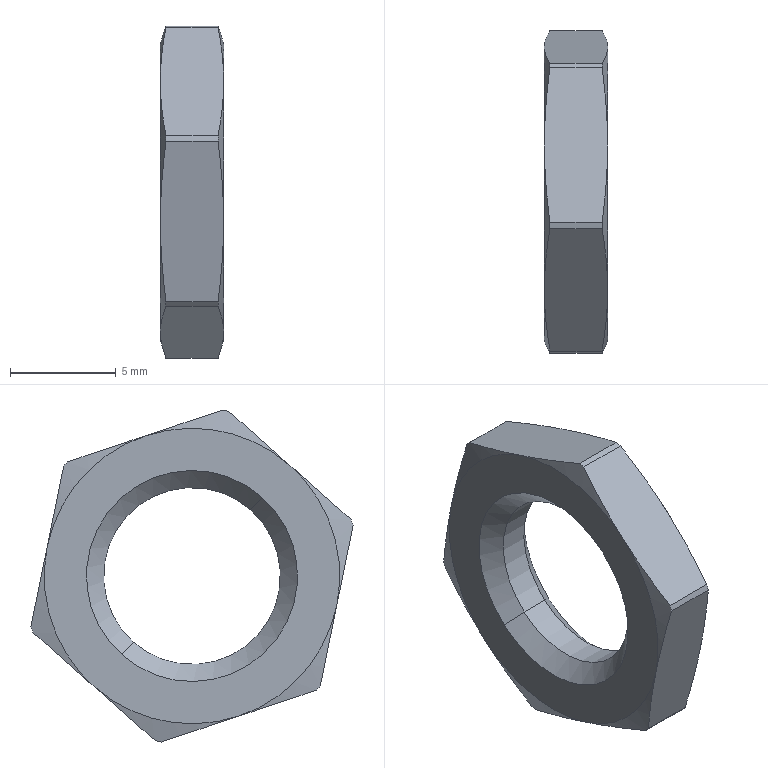Component | SolidWorks | SRK1010_nut_nut-1 | 1 solid | 32 faces | box 3 x 15.27 x 15.73 mm | volume 322 mm3 | cone 16 | cylinder 8 | plane 8 | commonest cylinder face diameters 16 x6 8.376 x2
STEP:
#1=COLOUR_RGB('',0.7922,0.8196,0.9333);
#2=FILL_AREA_STYLE_COLOUR('',#1);
#3=FILL_AREA_STYLE('',(#2));
#4=SURFACE_STYLE_FILL_AREA(#3);
#5=SURFACE_SIDE_STYLE('',(#4));
#6=SURFACE_STYLE_USAGE(.BOTH.,#5);
#7=PRESENTATION_STYLE_ASSIGNMENT((#6));
#8=CARTESIAN_POINT('',(-5.625,1.353,-4.032));
#9=VERTEX_POINT('',#8);
#10=CARTESIAN_POINT('',(-5.625,1.572,-4.278));
#11=VERTEX_POINT('',#10);
#12=CARTESIAN_POINT('',(-5.625,1.462,-4.155));
#13=DIRECTION('',(1.,-0.,-0.));
#14=DIRECTION('',(0.,0.6632,-0.7485));
#15=AXIS2_PLACEMENT_3D('',#12,#13,#14);
#16=CIRCLE('',#15,0.1649);
#17=EDGE_CURVE('',#9,#11,#16,.T.);
#18=ORIENTED_EDGE('',*,*,#17,.T.);
#19=CARTESIAN_POINT('',(-5.657,1.593,-4.302));
#20=VERTEX_POINT('',#19);
#21=CARTESIAN_POINT('',(-5.657,1.593,-4.302));
#22=DIRECTION('',(-0.7071,0.4689,-0.5292));
#23=VECTOR('',#22,39.37);
#24=LINE('',#21,#23);
#25=EDGE_CURVE('',#11,#20,#24,.T.);
#26=ORIENTED_EDGE('',*,*,#25,.T.);
#27=CARTESIAN_POINT('',(-5.657,1.332,-4.008));
#28=VERTEX_POINT('',#27);
#29=CARTESIAN_POINT('',(-5.657,1.462,-4.155));
#30=DIRECTION('',(1.,-0.,-0.));
#31=DIRECTION('',(0.,0.6632,-0.7485));
#32=AXIS2_PLACEMENT_3D('',#29,#30,#31);
#33=CIRCLE('',#32,0.1969);
#34=EDGE_CURVE('',#28,#20,#33,.T.);
#35=ORIENTED_EDGE('',*,*,#34,.F.);
#36=CARTESIAN_POINT('',(-5.657,1.332,-4.008));
#37=DIRECTION('',(-0.7071,-0.4689,0.5292));
#38=VECTOR('',#37,39.37);
#39=LINE('',#36,#38);
#40=EDGE_CURVE('',#9,#28,#39,.T.);
#41=ORIENTED_EDGE('',*,*,#40,.F.);
#42=EDGE_LOOP('',(#18,#26,#35,#41));
#43=FACE_OUTER_BOUND('',#42,.T.);
#44=CARTESIAN_POINT('',(-5.657,1.462,-4.155));
#45=DIRECTION('',(-1.,0.,0.));
#46=DIRECTION('',(0.,-0.6632,0.7485));
#47=AXIS2_PLACEMENT_3D('',#44,#45,#46);
#48=CONICAL_SURFACE('',#47,0.1969,0.7854);
#49=ADVANCED_FACE('',(#43),#48,.F.);
#50=ORIENTED_EDGE('',*,*,#17,.F.);
#51=CARTESIAN_POINT('',(-5.571,1.353,-4.032));
#52=VERTEX_POINT('',#51);
#53=CARTESIAN_POINT('',(-5.657,1.353,-4.032));
#54=DIRECTION('',(1.,-0.,-0.));
#55=VECTOR('',#54,39.37);
#56=LINE('',#53,#55);
#57=EDGE_CURVE('',#9,#52,#56,.T.);
#58=ORIENTED_EDGE('',*,*,#57,.T.);
#59=CARTESIAN_POINT('',(-5.571,1.572,-4.278));
#60=VERTEX_POINT('',#59);
#61=CARTESIAN_POINT('',(-5.571,1.462,-4.155));
#62=DIRECTION('',(1.,-0.,-0.));
#63=DIRECTION('',(0.,0.6632,-0.7485));
#64=AXIS2_PLACEMENT_3D('',#61,#62,#63);
#65=CIRCLE('',#64,0.1649);
#66=EDGE_CURVE('',#52,#60,#65,.T.);
#67=ORIENTED_EDGE('',*,*,#66,.T.);
#68=CARTESIAN_POINT('',(-5.657,1.572,-4.278));
#69=DIRECTION('',(1.,-0.,-0.));
#70=VECTOR('',#69,39.37);
#71=LINE('',#68,#70);
#72=EDGE_CURVE('',#11,#60,#71,.T.);
#73=ORIENTED_EDGE('',*,*,#72,.F.);
#74=EDGE_LOOP('',(#50,#58,#67,#73));
#75=FACE_OUTER_BOUND('',#74,.T.);
#76=CARTESIAN_POINT('',(-5.657,1.462,-4.155));
#77=DIRECTION('',(1.,-0.,-0.));
#78=DIRECTION('',(0.,0.6632,-0.7485));
#79=AXIS2_PLACEMENT_3D('',#76,#77,#78);
#80=CYLINDRICAL_SURFACE('',#79,0.1649);
#81=ADVANCED_FACE('',(#75),#80,.F.);
#82=ORIENTED_EDGE('',*,*,#66,.F.);
#83=CARTESIAN_POINT('',(-5.539,1.332,-4.008));
#84=VERTEX_POINT('',#83);
#85=CARTESIAN_POINT('',(-5.571,1.353,-4.032));
#86=DIRECTION('',(0.7071,-0.4689,0.5292));
#87=VECTOR('',#86,39.37);
#88=LINE('',#85,#87);
#89=EDGE_CURVE('',#52,#84,#88,.T.);
#90=ORIENTED_EDGE('',*,*,#89,.T.);
#91=CARTESIAN_POINT('',(-5.539,1.593,-4.302));
#92=VERTEX_POINT('',#91);
#93=CARTESIAN_POINT('',(-5.539,1.462,-4.155));
#94=DIRECTION('',(1.,-0.,-0.));
#95=DIRECTION('',(0.,0.6632,-0.7485));
#96=AXIS2_PLACEMENT_3D('',#93,#94,#95);
#97=CIRCLE('',#96,0.1969);
#98=EDGE_CURVE('',#84,#92,#97,.T.);
#99=ORIENTED_EDGE('',*,*,#98,.T.);
#100=CARTESIAN_POINT('',(-5.571,1.572,-4.278));
#101=DIRECTION('',(0.7071,0.4689,-0.5292));
#102=VECTOR('',#101,39.37);
#103=LINE('',#100,#102);
#104=EDGE_CURVE('',#60,#92,#103,.T.);
#105=ORIENTED_EDGE('',*,*,#104,.F.);
#106=EDGE_LOOP('',(#82,#90,#99,#105));
#107=FACE_OUTER_BOUND('',#106,.T.);
#108=CARTESIAN_POINT('',(-5.571,1.462,-4.155));
#109=DIRECTION('',(1.,-0.,-0.));
#110=DIRECTION('',(0.,0.6632,-0.7485));
#111=AXIS2_PLACEMENT_3D('',#108,#109,#110);
#112=CONICAL_SURFACE('',#111,0.1649,0.7854);
#113=ADVANCED_FACE('',(#107),#112,.F.);
#114=CARTESIAN_POINT('',(-5.539,1.645,-4.361));
#115=VERTEX_POINT('',#114);
#116=CARTESIAN_POINT('',(-5.539,1.732,-4.1));
#117=VERTEX_POINT('',#116);
#118=CARTESIAN_POINT('',(-5.539,1.462,-4.155));
#119=DIRECTION('',(1.,-0.,-0.));
#120=DIRECTION('',(0.,0.6632,-0.7485));
#121=AXIS2_PLACEMENT_3D('',#118,#119,#120);
#122=CIRCLE('',#121,0.2756);
#123=EDGE_CURVE('',#115,#117,#122,.T.);
#124=ORIENTED_EDGE('',*,*,#123,.T.);
#125=CARTESIAN_POINT('',(-5.539,1.549,-3.894));
#126=VERTEX_POINT('',#125);
#127=CARTESIAN_POINT('',(-5.539,1.462,-4.155));
#128=DIRECTION('',(1.,-0.,-0.));
#129=DIRECTION('',(0.,0.6632,-0.7485));
#130=AXIS2_PLACEMENT_3D('',#127,#128,#129);
#131=CIRCLE('',#130,0.2756);
#132=EDGE_CURVE('',#117,#126,#131,.T.);
#133=ORIENTED_EDGE('',*,*,#132,.T.);
#134=CARTESIAN_POINT('',(-5.539,1.279,-3.949));
#135=VERTEX_POINT('',#134);
#136=CARTESIAN_POINT('',(-5.539,1.462,-4.155));
#137=DIRECTION('',(1.,-0.,-0.));
#138=DIRECTION('',(0.,0.6632,-0.7485));
#139=AXIS2_PLACEMENT_3D('',#136,#137,#138);
#140=CIRCLE('',#139,0.2756);
#141=EDGE_CURVE('',#126,#135,#140,.T.);
#142=ORIENTED_EDGE('',*,*,#141,.T.);
#143=CARTESIAN_POINT('',(-5.539,1.192,-4.21));
#144=VERTEX_POINT('',#143);
#145=CARTESIAN_POINT('',(-5.539,1.462,-4.155));
#146=DIRECTION('',(1.,-0.,-0.));
#147=DIRECTION('',(0.,0.6632,-0.7485));
#148=AXIS2_PLACEMENT_3D('',#145,#146,#147);
#149=CIRCLE('',#148,0.2756);
#150=EDGE_CURVE('',#135,#144,#149,.T.);
#151=ORIENTED_EDGE('',*,*,#150,.T.);
#152=CARTESIAN_POINT('',(-5.539,1.375,-4.416));
#153=VERTEX_POINT('',#152);
#154=CARTESIAN_POINT('',(-5.539,1.462,-4.155));
#155=DIRECTION('',(1.,-0.,-0.));
#156=DIRECTION('',(0.,0.6632,-0.7485));
#157=AXIS2_PLACEMENT_3D('',#154,#155,#156);
#158=CIRCLE('',#157,0.2756);
#159=EDGE_CURVE('',#144,#153,#158,.T.);
#160=ORIENTED_EDGE('',*,*,#159,.T.);
#161=CARTESIAN_POINT('',(-5.539,1.462,-4.155));
#162=DIRECTION('',(1.,-0.,-0.));
#163=DIRECTION('',(0.,0.6632,-0.7485));
#164=AXIS2_PLACEMENT_3D('',#161,#162,#163);
#165=CIRCLE('',#164,0.2756);
#166=EDGE_CURVE('',#153,#115,#165,.T.);
#167=ORIENTED_EDGE('',*,*,#166,.T.);
#168=EDGE_LOOP('',(#124,#133,#142,#151,#160,#167));
#169=FACE_OUTER_BOUND('',#168,.T.);
#170=CARTESIAN_POINT('',(-5.539,1.462,-4.155));
#171=DIRECTION('',(1.,-0.,-0.));
#172=DIRECTION('',(0.,0.6632,-0.7485));
#173=AXIS2_PLACEMENT_3D('',#170,#171,#172);
#174=CIRCLE('',#173,0.1969);
#175=EDGE_CURVE('',#92,#84,#174,.T.);
#176=ORIENTED_EDGE('',*,*,#175,.F.);
#177=ORIENTED_EDGE('',*,*,#98,.F.);
#178=EDGE_LOOP('',(#176,#177));
#179=FACE_BOUND('',#178,.T.);
#180=CARTESIAN_POINT('',(-5.539,1.462,-4.155));
#181=DIRECTION('',(-1.,0.,0.));
#182=DIRECTION('',(-0.,-0.6632,0.7485));
#183=AXIS2_PLACEMENT_3D('',#180,#181,#182);
#184=PLANE('',#183);
#185=ADVANCED_FACE('',(#169,#179),#184,.F.);
#186=CARTESIAN_POINT('',(-5.657,1.645,-4.361));
#187=VERTEX_POINT('',#186);
#188=CARTESIAN_POINT('',(-5.657,1.732,-4.1));
#189=VERTEX_POINT('',#188);
#190=CARTESIAN_POINT('',(-5.657,1.462,-4.155));
#191=DIRECTION('',(1.,-0.,-0.));
#192=DIRECTION('',(0.,0.6632,-0.7485));
#193=AXIS2_PLACEMENT_3D('',#190,#191,#192);
#194=CIRCLE('',#193,0.2756);
#195=EDGE_CURVE('',#187,#189,#194,.T.);
#196=ORIENTED_EDGE('',*,*,#195,.F.);
#197=CARTESIAN_POINT('',(-5.657,1.375,-4.416));
#198=VERTEX_POINT('',#197);
#199=CARTESIAN_POINT('',(-5.657,1.462,-4.155));
#200=DIRECTION('',(1.,-0.,-0.));
#201=DIRECTION('',(0.,0.6632,-0.7485));
#202=AXIS2_PLACEMENT_3D('',#199,#200,#201);
#203=CIRCLE('',#202,0.2756);
#204=EDGE_CURVE('',#198,#187,#203,.T.);
#205=ORIENTED_EDGE('',*,*,#204,.F.);
#206=CARTESIAN_POINT('',(-5.657,1.192,-4.21));
#207=VERTEX_POINT('',#206);
#208=CARTESIAN_POINT('',(-5.657,1.462,-4.155));
#209=DIRECTION('',(1.,-0.,-0.));
#210=DIRECTION('',(0.,0.6632,-0.7485));
#211=AXIS2_PLACEMENT_3D('',#208,#209,#210);
#212=CIRCLE('',#211,0.2756);
#213=EDGE_CURVE('',#207,#198,#212,.T.);
#214=ORIENTED_EDGE('',*,*,#213,.F.);
#215=CARTESIAN_POINT('',(-5.657,1.279,-3.949));
#216=VERTEX_POINT('',#215);
#217=CARTESIAN_POINT('',(-5.657,1.462,-4.155));
#218=DIRECTION('',(1.,-0.,-0.));
#219=DIRECTION('',(0.,0.6632,-0.7485));
#220=AXIS2_PLACEMENT_3D('',#217,#218,#219);
#221=CIRCLE('',#220,0.2756);
#222=EDGE_CURVE('',#216,#207,#221,.T.);
#223=ORIENTED_EDGE('',*,*,#222,.F.);
#224=CARTESIAN_POINT('',(-5.657,1.549,-3.894));
#225=VERTEX_POINT('',#224);
#226=CARTESIAN_POINT('',(-5.657,1.462,-4.155));
#227=DIRECTION('',(1.,-0.,-0.));
#228=DIRECTION('',(0.,0.6632,-0.7485));
#229=AXIS2_PLACEMENT_3D('',#226,#227,#228);
#230=CIRCLE('',#229,0.2756);
#231=EDGE_CURVE('',#225,#216,#230,.T.);
#232=ORIENTED_EDGE('',*,*,#231,.F.);
#233=CARTESIAN_POINT('',(-5.657,1.462,-4.155));
#234=DIRECTION('',(1.,-0.,-0.));
#235=DIRECTION('',(0.,0.6632,-0.7485));
#236=AXIS2_PLACEMENT_3D('',#233,#234,#235);
#237=CIRCLE('',#236,0.2756);
#238=EDGE_CURVE('',#189,#225,#237,.T.);
#239=ORIENTED_EDGE('',*,*,#238,.F.);
#240=EDGE_LOOP('',(#196,#205,#214,#223,#232,#239));
#241=FACE_OUTER_BOUND('',#240,.T.);
#242=ORIENTED_EDGE('',*,*,#34,.T.);
#243=CARTESIAN_POINT('',(-5.657,1.462,-4.155));
#244=DIRECTION('',(1.,-0.,-0.));
#245=DIRECTION('',(0.,0.6632,-0.7485));
#246=AXIS2_PLACEMENT_3D('',#243,#244,#245);
#247=CIRCLE('',#246,0.1969);
#248=EDGE_CURVE('',#20,#28,#247,.T.);
#249=ORIENTED_EDGE('',*,*,#248,.T.);
#250=EDGE_LOOP('',(#242,#249));
#251=FACE_BOUND('',#250,.T.);
#252=CARTESIAN_POINT('',(-5.657,1.669,-3.972));
#253=DIRECTION('',(1.,-0.,-0.));
#254=DIRECTION('',(0.,0.6632,-0.7485));
#255=AXIS2_PLACEMENT_3D('',#252,#253,#254);
#256=PLANE('',#255);
#257=ADVANCED_FACE('',(#241,#251),#256,.F.);
#258=CARTESIAN_POINT('',(-5.55,1.223,-4.36));
#259=VERTEX_POINT('',#258);
#260=CARTESIAN_POINT('',(-5.55,1.223,-4.36));
#261=CARTESIAN_POINT('',(-5.543,1.213,-4.31));
#262=CARTESIAN_POINT('',(-5.539,1.202,-4.26));
#263=CARTESIAN_POINT('',(-5.539,1.192,-4.21));
#264=B_SPLINE_CURVE_WITH_KNOTS('',3,(#260,#261,#262,#263),.UNSPECIFIED.,.F.,.F.,(4,4),(0.00000154,0.003875),.UNSPECIFIED.);
#265=EDGE_CURVE('',#259,#144,#264,.T.);
#266=ORIENTED_EDGE('',*,*,#265,.F.);
#267=CARTESIAN_POINT('',(-5.55,1.23,-4.368));
#268=VERTEX_POINT('',#267);
#269=CARTESIAN_POINT('',(-5.55,1.462,-4.155));
#270=DIRECTION('',(1.,-0.,-0.));
#271=DIRECTION('',(0.,0.6632,-0.7485));
#272=AXIS2_PLACEMENT_3D('',#269,#270,#271);
#273=CIRCLE('',#272,0.315);
#274=EDGE_CURVE('',#259,#268,#273,.T.);
#275=ORIENTED_EDGE('',*,*,#274,.T.);
#276=CARTESIAN_POINT('',(-5.539,1.375,-4.416));
#277=CARTESIAN_POINT('',(-5.539,1.327,-4.4));
#278=CARTESIAN_POINT('',(-5.543,1.279,-4.384));
#279=CARTESIAN_POINT('',(-5.55,1.23,-4.368));
#280=B_SPLINE_CURVE_WITH_KNOTS('',3,(#276,#277,#278,#279),.UNSPECIFIED.,.F.,.F.,(4,4),(0.003875,0.007748),.UNSPECIFIED.);
#281=EDGE_CURVE('',#153,#268,#280,.T.);
#282=ORIENTED_EDGE('',*,*,#281,.F.);
#283=ORIENTED_EDGE('',*,*,#159,.F.);
#284=EDGE_LOOP('',(#266,#275,#282,#283));
#285=FACE_OUTER_BOUND('',#284,.T.);
#286=CARTESIAN_POINT('',(-5.55,1.462,-4.155));
#287=DIRECTION('',(-1.,0.,0.));
#288=DIRECTION('',(0.,-0.6632,0.7485));
#289=AXIS2_PLACEMENT_3D('',#286,#287,#288);
#290=CONICAL_SURFACE('',#289,0.315,1.309);
#291=ADVANCED_FACE('',(#285),#290,.T.);
#292=CARTESIAN_POINT('',(-5.55,1.162,-4.061));
#293=VERTEX_POINT('',#292);
#294=CARTESIAN_POINT('',(-5.539,1.192,-4.21));
#295=CARTESIAN_POINT('',(-5.539,1.182,-4.16));
#296=CARTESIAN_POINT('',(-5.543,1.172,-4.111));
#297=CARTESIAN_POINT('',(-5.55,1.162,-4.061));
#298=B_SPLINE_CURVE_WITH_KNOTS('',3,(#294,#295,#296,#297),.UNSPECIFIED.,.F.,.F.,(4,4),(0.003875,0.007748),.UNSPECIFIED.);
#299=EDGE_CURVE('',#144,#293,#298,.T.);
#300=ORIENTED_EDGE('',*,*,#299,.F.);
#301=ORIENTED_EDGE('',*,*,#150,.F.);
#302=CARTESIAN_POINT('',(-5.55,1.165,-4.05));
#303=VERTEX_POINT('',#302);
#304=CARTESIAN_POINT('',(-5.55,1.165,-4.05));
#305=CARTESIAN_POINT('',(-5.546,1.184,-4.033));
#306=CARTESIAN_POINT('',(-5.544,1.203,-4.016));
#307=CARTESIAN_POINT('',(-5.54,1.241,-3.982));
#308=CARTESIAN_POINT('',(-5.539,1.26,-3.966));
#309=CARTESIAN_POINT('',(-5.539,1.279,-3.949));
#310=B_SPLINE_CURVE_WITH_KNOTS('',3,(#304,#305,#306,#307,#308,#309),.UNSPECIFIED.,.F.,.F.,(4,2,4),(0.006929,0.008875,0.01082),.UNSPECIFIED.);
#311=EDGE_CURVE('',#303,#135,#310,.T.);
#312=ORIENTED_EDGE('',*,*,#311,.F.);
#313=CARTESIAN_POINT('',(-5.55,1.462,-4.155));
#314=DIRECTION('',(1.,-0.,-0.));
#315=DIRECTION('',(0.,0.6632,-0.7485));
#316=AXIS2_PLACEMENT_3D('',#313,#314,#315);
#317=CIRCLE('',#316,0.315);
#318=EDGE_CURVE('',#303,#293,#317,.T.);
#319=ORIENTED_EDGE('',*,*,#318,.T.);
#320=EDGE_LOOP('',(#300,#301,#312,#319));
#321=FACE_OUTER_BOUND('',#320,.T.);
#322=CARTESIAN_POINT('',(-5.55,1.462,-4.155));
#323=DIRECTION('',(-1.,0.,0.));
#324=DIRECTION('',(0.,-0.6632,0.7485));
#325=AXIS2_PLACEMENT_3D('',#322,#323,#324);
#326=CONICAL_SURFACE('',#325,0.315,1.309);
#327=ADVANCED_FACE('',(#321),#326,.T.);
#328=CARTESIAN_POINT('',(-5.55,1.394,-3.848));
#329=VERTEX_POINT('',#328);
#330=CARTESIAN_POINT('',(-5.539,1.279,-3.949));
#331=CARTESIAN_POINT('',(-5.539,1.318,-3.915));
#332=CARTESIAN_POINT('',(-5.543,1.356,-3.881));
#333=CARTESIAN_POINT('',(-5.55,1.394,-3.848));
#334=B_SPLINE_CURVE_WITH_KNOTS('',3,(#330,#331,#332,#333),.UNSPECIFIED.,.F.,.F.,(4,4),(0.01082,0.01473),.UNSPECIFIED.);
#335=EDGE_CURVE('',#135,#329,#334,.T.);
#336=ORIENTED_EDGE('',*,*,#335,.F.);
#337=ORIENTED_EDGE('',*,*,#141,.F.);
#338=CARTESIAN_POINT('',(-5.55,1.405,-3.845));
#339=VERTEX_POINT('',#338);
#340=CARTESIAN_POINT('',(-5.55,1.405,-3.845));
#341=CARTESIAN_POINT('',(-5.543,1.453,-3.861));
#342=CARTESIAN_POINT('',(-5.539,1.501,-3.877));
#343=CARTESIAN_POINT('',(-5.539,1.549,-3.894));
#344=B_SPLINE_CURVE_WITH_KNOTS('',3,(#340,#341,#342,#343),.UNSPECIFIED.,.F.,.F.,(4,4),(0.00000154,0.003875),.UNSPECIFIED.);
#345=EDGE_CURVE('',#339,#126,#344,.T.);
#346=ORIENTED_EDGE('',*,*,#345,.F.);
#347=CARTESIAN_POINT('',(-5.55,1.462,-4.155));
#348=DIRECTION('',(1.,-0.,-0.));
#349=DIRECTION('',(0.,0.6632,-0.7485));
#350=AXIS2_PLACEMENT_3D('',#347,#348,#349);
#351=CIRCLE('',#350,0.315);
#352=EDGE_CURVE('',#339,#329,#351,.T.);
#353=ORIENTED_EDGE('',*,*,#352,.T.);
#354=EDGE_LOOP('',(#336,#337,#346,#353));
#355=FACE_OUTER_BOUND('',#354,.T.);
#356=CARTESIAN_POINT('',(-5.55,1.462,-4.155));
#357=DIRECTION('',(-1.,0.,0.));
#358=DIRECTION('',(0.,-0.6632,0.7485));
#359=AXIS2_PLACEMENT_3D('',#356,#357,#358);
#360=CONICAL_SURFACE('',#359,0.315,1.309);
#361=ADVANCED_FACE('',(#355),#360,.T.);
#362=CARTESIAN_POINT('',(-5.55,1.694,-3.942));
#363=VERTEX_POINT('',#362);
#364=CARTESIAN_POINT('',(-5.539,1.549,-3.894));
#365=CARTESIAN_POINT('',(-5.539,1.598,-3.91));
#366=CARTESIAN_POINT('',(-5.543,1.646,-3.926));
#367=CARTESIAN_POINT('',(-5.55,1.694,-3.942));
#368=B_SPLINE_CURVE_WITH_KNOTS('',3,(#364,#365,#366,#367),.UNSPECIFIED.,.F.,.F.,(4,4),(0.003875,0.007748),.UNSPECIFIED.);
#369=EDGE_CURVE('',#126,#363,#368,.T.);
#370=ORIENTED_EDGE('',*,*,#369,.F.);
#371=ORIENTED_EDGE('',*,*,#132,.F.);
#372=CARTESIAN_POINT('',(-5.55,1.702,-3.95));
#373=VERTEX_POINT('',#372);
#374=CARTESIAN_POINT('',(-5.55,1.702,-3.95));
#375=CARTESIAN_POINT('',(-5.543,1.712,-4.));
#376=CARTESIAN_POINT('',(-5.539,1.722,-4.05));
#377=CARTESIAN_POINT('',(-5.539,1.732,-4.1));
#378=B_SPLINE_CURVE_WITH_KNOTS('',3,(#374,#375,#376,#377),.UNSPECIFIED.,.F.,.F.,(4,4),(0.00000154,0.003875),.UNSPECIFIED.);
#379=EDGE_CURVE('',#373,#117,#378,.T.);
#380=ORIENTED_EDGE('',*,*,#379,.F.);
#381=CARTESIAN_POINT('',(-5.55,1.462,-4.155));
#382=DIRECTION('',(1.,-0.,-0.));
#383=DIRECTION('',(0.,0.6632,-0.7485));
#384=AXIS2_PLACEMENT_3D('',#381,#382,#383);
#385=CIRCLE('',#384,0.315);
#386=EDGE_CURVE('',#373,#363,#385,.T.);
#387=ORIENTED_EDGE('',*,*,#386,.T.);
#388=EDGE_LOOP('',(#370,#371,#380,#387));
#389=FACE_OUTER_BOUND('',#388,.T.);
#390=CARTESIAN_POINT('',(-5.55,1.462,-4.155));
#391=DIRECTION('',(-1.,0.,0.));
#392=DIRECTION('',(0.,-0.6632,0.7485));
#393=AXIS2_PLACEMENT_3D('',#390,#391,#392);
#394=CONICAL_SURFACE('',#393,0.315,1.309);
#395=ADVANCED_FACE('',(#389),#394,.T.);
#396=CARTESIAN_POINT('',(-5.55,1.763,-4.249));
#397=VERTEX_POINT('',#396);
#398=CARTESIAN_POINT('',(-5.539,1.732,-4.1));
#399=CARTESIAN_POINT('',(-5.539,1.742,-4.15));
#400=CARTESIAN_POINT('',(-5.543,1.753,-4.199));
#401=CARTESIAN_POINT('',(-5.55,1.763,-4.249));
#402=B_SPLINE_CURVE_WITH_KNOTS('',3,(#398,#399,#400,#401),.UNSPECIFIED.,.F.,.F.,(4,4),(0.003875,0.007748),.UNSPECIFIED.);
#403=EDGE_CURVE('',#117,#397,#402,.T.);
#404=ORIENTED_EDGE('',*,*,#403,.F.);
#405=ORIENTED_EDGE('',*,*,#123,.F.);
#406=CARTESIAN_POINT('',(-5.55,1.759,-4.26));
#407=VERTEX_POINT('',#406);
#408=CARTESIAN_POINT('',(-5.55,1.759,-4.26));
#409=CARTESIAN_POINT('',(-5.543,1.721,-4.294));
#410=CARTESIAN_POINT('',(-5.539,1.683,-4.327));
#411=CARTESIAN_POINT('',(-5.539,1.645,-4.361));
#412=B_SPLINE_CURVE_WITH_KNOTS('',3,(#408,#409,#410,#411),.UNSPECIFIED.,.F.,.F.,(4,4),(0.01554,0.01944),.UNSPECIFIED.);
#413=EDGE_CURVE('',#407,#115,#412,.T.);
#414=ORIENTED_EDGE('',*,*,#413,.F.);
#415=CARTESIAN_POINT('',(-5.55,1.462,-4.155));
#416=DIRECTION('',(1.,-0.,-0.));
#417=DIRECTION('',(0.,0.6632,-0.7485));
#418=AXIS2_PLACEMENT_3D('',#415,#416,#417);
#419=CIRCLE('',#418,0.315);
#420=EDGE_CURVE('',#407,#397,#419,.T.);
#421=ORIENTED_EDGE('',*,*,#420,.T.);
#422=EDGE_LOOP('',(#404,#405,#414,#421));
#423=FACE_OUTER_BOUND('',#422,.T.);
#424=CARTESIAN_POINT('',(-5.55,1.462,-4.155));
#425=DIRECTION('',(-1.,0.,0.));
#426=DIRECTION('',(0.,-0.6632,0.7485));
#427=AXIS2_PLACEMENT_3D('',#424,#425,#426);
#428=CONICAL_SURFACE('',#427,0.315,1.309);
#429=ADVANCED_FACE('',(#423),#428,.T.);
#430=CARTESIAN_POINT('',(-5.55,1.531,-4.462));
#431=VERTEX_POINT('',#430);
#432=CARTESIAN_POINT('',(-5.539,1.645,-4.361));
#433=CARTESIAN_POINT('',(-5.539,1.626,-4.378));
#434=CARTESIAN_POINT('',(-5.54,1.607,-4.395));
#435=CARTESIAN_POINT('',(-5.544,1.569,-4.429));
#436=CARTESIAN_POINT('',(-5.546,1.55,-4.446));
#437=CARTESIAN_POINT('',(-5.55,1.531,-4.462));
#438=B_SPLINE_CURVE_WITH_KNOTS('',3,(#432,#433,#434,#435,#436,#437),.UNSPECIFIED.,.F.,.F.,(4,2,4),(0.01944,0.02138,0.02332),.UNSPECIFIED.);
#439=EDGE_CURVE('',#115,#431,#438,.T.);
#440=ORIENTED_EDGE('',*,*,#439,.F.);
#441=ORIENTED_EDGE('',*,*,#166,.F.);
#442=CARTESIAN_POINT('',(-5.55,1.52,-4.465));
#443=VERTEX_POINT('',#442);
#444=CARTESIAN_POINT('',(-5.55,1.52,-4.465));
#445=CARTESIAN_POINT('',(-5.543,1.471,-4.449));
#446=CARTESIAN_POINT('',(-5.539,1.423,-4.432));
#447=CARTESIAN_POINT('',(-5.539,1.375,-4.416));
#448=B_SPLINE_CURVE_WITH_KNOTS('',3,(#444,#445,#446,#447),.UNSPECIFIED.,.F.,.F.,(4,4),(0.00000154,0.003875),.UNSPECIFIED.);
#449=EDGE_CURVE('',#443,#153,#448,.T.);
#450=ORIENTED_EDGE('',*,*,#449,.F.);
#451=CARTESIAN_POINT('',(-5.55,1.462,-4.155));
#452=DIRECTION('',(1.,-0.,-0.));
#453=DIRECTION('',(0.,0.6632,-0.7485));
#454=AXIS2_PLACEMENT_3D('',#451,#452,#453);
#455=CIRCLE('',#454,0.315);
#456=EDGE_CURVE('',#443,#431,#455,.T.);
#457=ORIENTED_EDGE('',*,*,#456,.T.);
#458=EDGE_LOOP('',(#440,#441,#450,#457));
#459=FACE_OUTER_BOUND('',#458,.T.);
#460=CARTESIAN_POINT('',(-5.55,1.462,-4.155));
#461=DIRECTION('',(-1.,0.,0.));
#462=DIRECTION('',(0.,-0.6632,0.7485));
#463=AXIS2_PLACEMENT_3D('',#460,#461,#462);
#464=CONICAL_SURFACE('',#463,0.315,1.309);
#465=ADVANCED_FACE('',(#459),#464,.T.);
#466=CARTESIAN_POINT('',(-5.647,1.223,-4.36));
#467=VERTEX_POINT('',#466);
#468=CARTESIAN_POINT('',(-5.657,1.223,-4.36));
#469=DIRECTION('',(1.,-0.,-0.));
#470=VECTOR('',#469,39.37);
#471=LINE('',#468,#470);
#472=EDGE_CURVE('',#467,#259,#471,.T.);
#473=ORIENTED_EDGE('',*,*,#472,.F.);
#474=CARTESIAN_POINT('',(-5.647,1.23,-4.368));
#475=VERTEX_POINT('',#474);
#476=CARTESIAN_POINT('',(-5.647,1.462,-4.155));
#477=DIRECTION('',(1.,-0.,-0.));
#478=DIRECTION('',(0.,0.6632,-0.7485));
#479=AXIS2_PLACEMENT_3D('',#476,#477,#478);
#480=CIRCLE('',#479,0.315);
#481=EDGE_CURVE('',#467,#475,#480,.T.);
#482=ORIENTED_EDGE('',*,*,#481,.T.);
#483=CARTESIAN_POINT('',(-5.657,1.23,-4.368));
#484=DIRECTION('',(-1.,0.,0.));
#485=VECTOR('',#484,39.37);
#486=LINE('',#483,#485);
#487=EDGE_CURVE('',#268,#475,#486,.T.);
#488=ORIENTED_EDGE('',*,*,#487,.F.);
#489=ORIENTED_EDGE('',*,*,#274,.F.);
#490=EDGE_LOOP('',(#473,#482,#488,#489));
#491=FACE_OUTER_BOUND('',#490,.T.);
#492=CARTESIAN_POINT('',(-5.657,1.462,-4.155));
#493=DIRECTION('',(1.,-0.,-0.));
#494=DIRECTION('',(0.,0.6632,-0.7485));
#495=AXIS2_PLACEMENT_3D('',#492,#493,#494);
#496=CYLINDRICAL_SURFACE('',#495,0.315);
#497=ADVANCED_FACE('',(#491),#496,.T.);
#498=CARTESIAN_POINT('',(-5.647,1.162,-4.061));
#499=VERTEX_POINT('',#498);
#500=CARTESIAN_POINT('',(-5.657,1.162,-4.061));
#501=DIRECTION('',(-1.,0.,0.));
#502=VECTOR('',#501,39.37);
#503=LINE('',#500,#502);
#504=EDGE_CURVE('',#293,#499,#503,.T.);
#505=ORIENTED_EDGE('',*,*,#504,.F.);
#506=ORIENTED_EDGE('',*,*,#318,.F.);
#507=CARTESIAN_POINT('',(-5.647,1.165,-4.05));
#508=VERTEX_POINT('',#507);
#509=CARTESIAN_POINT('',(-5.657,1.165,-4.05));
#510=DIRECTION('',(1.,-0.,-0.));
#511=VECTOR('',#510,39.37);
#512=LINE('',#509,#511);
#513=EDGE_CURVE('',#508,#303,#512,.T.);
#514=ORIENTED_EDGE('',*,*,#513,.F.);
#515=CARTESIAN_POINT('',(-5.647,1.462,-4.155));
#516=DIRECTION('',(1.,-0.,-0.));
#517=DIRECTION('',(0.,0.6632,-0.7485));
#518=AXIS2_PLACEMENT_3D('',#515,#516,#517);
#519=CIRCLE('',#518,0.315);
#520=EDGE_CURVE('',#508,#499,#519,.T.);
#521=ORIENTED_EDGE('',*,*,#520,.T.);
#522=EDGE_LOOP('',(#505,#506,#514,#521));
#523=FACE_OUTER_BOUND('',#522,.T.);
#524=CARTESIAN_POINT('',(-5.657,1.462,-4.155));
#525=DIRECTION('',(1.,-0.,-0.));
#526=DIRECTION('',(0.,0.6632,-0.7485));
#527=AXIS2_PLACEMENT_3D('',#524,#525,#526);
#528=CYLINDRICAL_SURFACE('',#527,0.315);
#529=ADVANCED_FACE('',(#523),#528,.T.);
#530=CARTESIAN_POINT('',(-5.647,1.394,-3.848));
#531=VERTEX_POINT('',#530);
#532=CARTESIAN_POINT('',(-5.657,1.394,-3.848));
#533=DIRECTION('',(-1.,0.,0.));
#534=VECTOR('',#533,39.37);
#535=LINE('',#532,#534);
#536=EDGE_CURVE('',#329,#531,#535,.T.);
#537=ORIENTED_EDGE('',*,*,#536,.F.);
#538=ORIENTED_EDGE('',*,*,#352,.F.);
#539=CARTESIAN_POINT('',(-5.647,1.405,-3.845));
#540=VERTEX_POINT('',#539);
#541=CARTESIAN_POINT('',(-5.657,1.405,-3.845));
#542=DIRECTION('',(1.,-0.,-0.));
#543=VECTOR('',#542,39.37);
#544=LINE('',#541,#543);
#545=EDGE_CURVE('',#540,#339,#544,.T.);
#546=ORIENTED_EDGE('',*,*,#545,.F.);
#547=CARTESIAN_POINT('',(-5.647,1.462,-4.155));
#548=DIRECTION('',(1.,-0.,-0.));
#549=DIRECTION('',(0.,0.6632,-0.7485));
#550=AXIS2_PLACEMENT_3D('',#547,#548,#549);
#551=CIRCLE('',#550,0.315);
#552=EDGE_CURVE('',#540,#531,#551,.T.);
#553=ORIENTED_EDGE('',*,*,#552,.T.);
#554=EDGE_LOOP('',(#537,#538,#546,#553));
#555=FACE_OUTER_BOUND('',#554,.T.);
#556=CARTESIAN_POINT('',(-5.657,1.462,-4.155));
#557=DIRECTION('',(1.,-0.,-0.));
#558=DIRECTION('',(0.,0.6632,-0.7485));
#559=AXIS2_PLACEMENT_3D('',#556,#557,#558);
#560=CYLINDRICAL_SURFACE('',#559,0.315);
#561=ADVANCED_FACE('',(#555),#560,.T.);
#562=CARTESIAN_POINT('',(-5.647,1.694,-3.942));
#563=VERTEX_POINT('',#562);
#564=CARTESIAN_POINT('',(-5.657,1.694,-3.942));
#565=DIRECTION('',(-1.,0.,0.));
#566=VECTOR('',#565,39.37);
#567=LINE('',#564,#566);
#568=EDGE_CURVE('',#363,#563,#567,.T.);
#569=ORIENTED_EDGE('',*,*,#568,.F.);
#570=ORIENTED_EDGE('',*,*,#386,.F.);
#571=CARTESIAN_POINT('',(-5.647,1.702,-3.95));
#572=VERTEX_POINT('',#571);
#573=CARTESIAN_POINT('',(-5.657,1.702,-3.95));
#574=DIRECTION('',(1.,-0.,-0.));
#575=VECTOR('',#574,39.37);
#576=LINE('',#573,#575);
#577=EDGE_CURVE('',#572,#373,#576,.T.);
#578=ORIENTED_EDGE('',*,*,#577,.F.);
#579=CARTESIAN_POINT('',(-5.647,1.462,-4.155));
#580=DIRECTION('',(1.,-0.,-0.));
#581=DIRECTION('',(0.,0.6632,-0.7485));
#582=AXIS2_PLACEMENT_3D('',#579,#580,#581);
#583=CIRCLE('',#582,0.315);
#584=EDGE_CURVE('',#572,#563,#583,.T.);
#585=ORIENTED_EDGE('',*,*,#584,.T.);
#586=EDGE_LOOP('',(#569,#570,#578,#585));
#587=FACE_OUTER_BOUND('',#586,.T.);
#588=CARTESIAN_POINT('',(-5.657,1.462,-4.155));
#589=DIRECTION('',(1.,-0.,-0.));
#590=DIRECTION('',(0.,0.6632,-0.7485));
#591=AXIS2_PLACEMENT_3D('',#588,#589,#590);
#592=CYLINDRICAL_SURFACE('',#591,0.315);
#593=ADVANCED_FACE('',(#587),#592,.T.);
#594=CARTESIAN_POINT('',(-5.647,1.763,-4.249));
#595=VERTEX_POINT('',#594);
#596=CARTESIAN_POINT('',(-5.657,1.763,-4.249));
#597=DIRECTION('',(-1.,0.,0.));
#598=VECTOR('',#597,39.37);
#599=LINE('',#596,#598);
#600=EDGE_CURVE('',#397,#595,#599,.T.);
#601=ORIENTED_EDGE('',*,*,#600,.F.);
#602=ORIENTED_EDGE('',*,*,#420,.F.);
#603=CARTESIAN_POINT('',(-5.647,1.759,-4.26));
#604=VERTEX_POINT('',#603);
#605=CARTESIAN_POINT('',(-5.657,1.759,-4.26));
#606=DIRECTION('',(1.,-0.,-0.));
#607=VECTOR('',#606,39.37);
#608=LINE('',#605,#607);
#609=EDGE_CURVE('',#604,#407,#608,.T.);
#610=ORIENTED_EDGE('',*,*,#609,.F.);
#611=CARTESIAN_POINT('',(-5.647,1.462,-4.155));
#612=DIRECTION('',(1.,-0.,-0.));
#613=DIRECTION('',(0.,0.6632,-0.7485));
#614=AXIS2_PLACEMENT_3D('',#611,#612,#613);
#615=CIRCLE('',#614,0.315);
#616=EDGE_CURVE('',#604,#595,#615,.T.);
#617=ORIENTED_EDGE('',*,*,#616,.T.);
#618=EDGE_LOOP('',(#601,#602,#610,#617));
#619=FACE_OUTER_BOUND('',#618,.T.);
#620=CARTESIAN_POINT('',(-5.657,1.462,-4.155));
#621=DIRECTION('',(1.,-0.,-0.));
#622=DIRECTION('',(0.,0.6632,-0.7485));
#623=AXIS2_PLACEMENT_3D('',#620,#621,#622);
#624=CYLINDRICAL_SURFACE('',#623,0.315);
#625=ADVANCED_FACE('',(#619),#624,.T.);
#626=CARTESIAN_POINT('',(-5.647,1.531,-4.462));
#627=VERTEX_POINT('',#626);
#628=CARTESIAN_POINT('',(-5.657,1.531,-4.462));
#629=DIRECTION('',(-1.,0.,0.));
#630=VECTOR('',#629,39.37);
#631=LINE('',#628,#630);
#632=EDGE_CURVE('',#431,#627,#631,.T.);
#633=ORIENTED_EDGE('',*,*,#632,.F.);
#634=ORIENTED_EDGE('',*,*,#456,.F.);
#635=CARTESIAN_POINT('',(-5.647,1.52,-4.465));
#636=VERTEX_POINT('',#635);
#637=CARTESIAN_POINT('',(-5.657,1.52,-4.465));
#638=DIRECTION('',(1.,-0.,-0.));
#639=VECTOR('',#638,39.37);
#640=LINE('',#637,#639);
#641=EDGE_CURVE('',#636,#443,#640,.T.);
#642=ORIENTED_EDGE('',*,*,#641,.F.);
#643=CARTESIAN_POINT('',(-5.647,1.462,-4.155));
#644=DIRECTION('',(1.,-0.,-0.));
#645=DIRECTION('',(0.,0.6632,-0.7485));
#646=AXIS2_PLACEMENT_3D('',#643,#644,#645);
#647=CIRCLE('',#646,0.315);
#648=EDGE_CURVE('',#636,#627,#647,.T.);
#649=ORIENTED_EDGE('',*,*,#648,.T.);
#650=EDGE_LOOP('',(#633,#634,#642,#649));
#651=FACE_OUTER_BOUND('',#650,.T.);
#652=CARTESIAN_POINT('',(-5.657,1.462,-4.155));
#653=DIRECTION('',(1.,-0.,-0.));
#654=DIRECTION('',(0.,0.6632,-0.7485));
#655=AXIS2_PLACEMENT_3D('',#652,#653,#654);
#656=CYLINDRICAL_SURFACE('',#655,0.315);
#657=ADVANCED_FACE('',(#651),#656,.T.);
#658=CARTESIAN_POINT('',(-5.647,1.162,-4.061));
#659=CARTESIAN_POINT('',(-5.653,1.172,-4.111));
#660=CARTESIAN_POINT('',(-5.657,1.182,-4.16));
#661=CARTESIAN_POINT('',(-5.657,1.192,-4.21));
#662=B_SPLINE_CURVE_WITH_KNOTS('',3,(#658,#659,#660,#661),.UNSPECIFIED.,.F.,.F.,(4,4),(0.00000154,0.003875),.UNSPECIFIED.);
#663=EDGE_CURVE('',#499,#207,#662,.T.);
#664=ORIENTED_EDGE('',*,*,#663,.F.);
#665=ORIENTED_EDGE('',*,*,#520,.F.);
#666=CARTESIAN_POINT('',(-5.657,1.279,-3.949));
#667=CARTESIAN_POINT('',(-5.657,1.26,-3.966));
#668=CARTESIAN_POINT('',(-5.656,1.241,-3.982));
#669=CARTESIAN_POINT('',(-5.653,1.203,-4.016));
#670=CARTESIAN_POINT('',(-5.65,1.184,-4.033));
#671=CARTESIAN_POINT('',(-5.647,1.165,-4.05));
#672=B_SPLINE_CURVE_WITH_KNOTS('',3,(#666,#667,#668,#669,#670,#671),.UNSPECIFIED.,.F.,.F.,(4,2,4),(0.01944,0.02138,0.02332),.UNSPECIFIED.);
#673=EDGE_CURVE('',#216,#508,#672,.T.);
#674=ORIENTED_EDGE('',*,*,#673,.F.);
#675=ORIENTED_EDGE('',*,*,#222,.T.);
#676=EDGE_LOOP('',(#664,#665,#674,#675));
#677=FACE_OUTER_BOUND('',#676,.T.);
#678=CARTESIAN_POINT('',(-5.657,1.462,-4.155));
#679=DIRECTION('',(1.,-0.,-0.));
#680=DIRECTION('',(0.,0.6632,-0.7485));
#681=AXIS2_PLACEMENT_3D('',#678,#679,#680);
#682=CONICAL_SURFACE('',#681,0.2756,1.309);
#683=ADVANCED_FACE('',(#677),#682,.T.);
#684=CARTESIAN_POINT('',(-5.657,1.192,-4.21));
#685=CARTESIAN_POINT('',(-5.657,1.202,-4.26));
#686=CARTESIAN_POINT('',(-5.653,1.213,-4.31));
#687=CARTESIAN_POINT('',(-5.647,1.223,-4.36));
#688=B_SPLINE_CURVE_WITH_KNOTS('',3,(#684,#685,#686,#687),.UNSPECIFIED.,.F.,.F.,(4,4),(0.003875,0.007748),.UNSPECIFIED.);
#689=EDGE_CURVE('',#207,#467,#688,.T.);
#690=ORIENTED_EDGE('',*,*,#689,.F.);
#691=ORIENTED_EDGE('',*,*,#213,.T.);
#692=CARTESIAN_POINT('',(-5.647,1.23,-4.368));
#693=CARTESIAN_POINT('',(-5.653,1.279,-4.384));
#694=CARTESIAN_POINT('',(-5.657,1.327,-4.4));
#695=CARTESIAN_POINT('',(-5.657,1.375,-4.416));
#696=B_SPLINE_CURVE_WITH_KNOTS('',3,(#692,#693,#694,#695),.UNSPECIFIED.,.F.,.F.,(4,4),(0.00000154,0.003875),.UNSPECIFIED.);
#697=EDGE_CURVE('',#475,#198,#696,.T.);
#698=ORIENTED_EDGE('',*,*,#697,.F.);
#699=ORIENTED_EDGE('',*,*,#481,.F.);
#700=EDGE_LOOP('',(#690,#691,#698,#699));
#701=FACE_OUTER_BOUND('',#700,.T.);
#702=CARTESIAN_POINT('',(-5.657,1.462,-4.155));
#703=DIRECTION('',(1.,-0.,-0.));
#704=DIRECTION('',(0.,0.6632,-0.7485));
#705=AXIS2_PLACEMENT_3D('',#702,#703,#704);
#706=CONICAL_SURFACE('',#705,0.2756,1.309);
#707=ADVANCED_FACE('',(#701),#706,.T.);
#708=CARTESIAN_POINT('',(-5.647,1.394,-3.848));
#709=CARTESIAN_POINT('',(-5.653,1.356,-3.881));
#710=CARTESIAN_POINT('',(-5.657,1.318,-3.915));
#711=CARTESIAN_POINT('',(-5.657,1.279,-3.949));
#712=B_SPLINE_CURVE_WITH_KNOTS('',3,(#708,#709,#710,#711),.UNSPECIFIED.,.F.,.F.,(4,4),(0.01554,0.01944),.UNSPECIFIED.);
#713=EDGE_CURVE('',#531,#216,#712,.T.);
#714=ORIENTED_EDGE('',*,*,#713,.F.);
#715=ORIENTED_EDGE('',*,*,#552,.F.);
#716=CARTESIAN_POINT('',(-5.657,1.549,-3.894));
#717=CARTESIAN_POINT('',(-5.657,1.501,-3.877));
#718=CARTESIAN_POINT('',(-5.653,1.453,-3.861));
#719=CARTESIAN_POINT('',(-5.647,1.405,-3.845));
#720=B_SPLINE_CURVE_WITH_KNOTS('',3,(#716,#717,#718,#719),.UNSPECIFIED.,.F.,.F.,(4,4),(0.003875,0.007748),.UNSPECIFIED.);
#721=EDGE_CURVE('',#225,#540,#720,.T.);
#722=ORIENTED_EDGE('',*,*,#721,.F.);
#723=ORIENTED_EDGE('',*,*,#231,.T.);
#724=EDGE_LOOP('',(#714,#715,#722,#723));
#725=FACE_OUTER_BOUND('',#724,.T.);
#726=CARTESIAN_POINT('',(-5.657,1.462,-4.155));
#727=DIRECTION('',(1.,-0.,-0.));
#728=DIRECTION('',(0.,0.6632,-0.7485));
#729=AXIS2_PLACEMENT_3D('',#726,#727,#728);
#730=CONICAL_SURFACE('',#729,0.2756,1.309);
#731=ADVANCED_FACE('',(#725),#730,.T.);
#732=CARTESIAN_POINT('',(-5.647,1.694,-3.942));
#733=CARTESIAN_POINT('',(-5.653,1.646,-3.926));
#734=CARTESIAN_POINT('',(-5.657,1.598,-3.91));
#735=CARTESIAN_POINT('',(-5.657,1.549,-3.894));
#736=B_SPLINE_CURVE_WITH_KNOTS('',3,(#732,#733,#734,#735),.UNSPECIFIED.,.F.,.F.,(4,4),(0.00000154,0.003875),.UNSPECIFIED.);
#737=EDGE_CURVE('',#563,#225,#736,.T.);
#738=ORIENTED_EDGE('',*,*,#737,.F.);
#739=ORIENTED_EDGE('',*,*,#584,.F.);
#740=CARTESIAN_POINT('',(-5.657,1.732,-4.1));
#741=CARTESIAN_POINT('',(-5.657,1.722,-4.05));
#742=CARTESIAN_POINT('',(-5.653,1.712,-4.));
#743=CARTESIAN_POINT('',(-5.647,1.702,-3.95));
#744=B_SPLINE_CURVE_WITH_KNOTS('',3,(#740,#741,#742,#743),.UNSPECIFIED.,.F.,.F.,(4,4),(0.003875,0.007748),.UNSPECIFIED.);
#745=EDGE_CURVE('',#189,#572,#744,.T.);
#746=ORIENTED_EDGE('',*,*,#745,.F.);
#747=ORIENTED_EDGE('',*,*,#238,.T.);
#748=EDGE_LOOP('',(#738,#739,#746,#747));
#749=FACE_OUTER_BOUND('',#748,.T.);
#750=CARTESIAN_POINT('',(-5.657,1.462,-4.155));
#751=DIRECTION('',(1.,-0.,-0.));
#752=DIRECTION('',(0.,0.6632,-0.7485));
#753=AXIS2_PLACEMENT_3D('',#750,#751,#752);
#754=CONICAL_SURFACE('',#753,0.2756,1.309);
#755=ADVANCED_FACE('',(#749),#754,.T.);
#756=CARTESIAN_POINT('',(-5.647,1.763,-4.249));
#757=CARTESIAN_POINT('',(-5.653,1.753,-4.199));
#758=CARTESIAN_POINT('',(-5.657,1.742,-4.15));
#759=CARTESIAN_POINT('',(-5.657,1.732,-4.1));
#760=B_SPLINE_CURVE_WITH_KNOTS('',3,(#756,#757,#758,#759),.UNSPECIFIED.,.F.,.F.,(4,4),(0.00000154,0.003875),.UNSPECIFIED.);
#761=EDGE_CURVE('',#595,#189,#760,.T.);
#762=ORIENTED_EDGE('',*,*,#761,.F.);
#763=ORIENTED_EDGE('',*,*,#616,.F.);
#764=CARTESIAN_POINT('',(-5.657,1.645,-4.361));
#765=CARTESIAN_POINT('',(-5.657,1.683,-4.327));
#766=CARTESIAN_POINT('',(-5.653,1.721,-4.294));
#767=CARTESIAN_POINT('',(-5.647,1.759,-4.26));
#768=B_SPLINE_CURVE_WITH_KNOTS('',3,(#764,#765,#766,#767),.UNSPECIFIED.,.F.,.F.,(4,4),(0.01082,0.01473),.UNSPECIFIED.);
#769=EDGE_CURVE('',#187,#604,#768,.T.);
#770=ORIENTED_EDGE('',*,*,#769,.F.);
#771=ORIENTED_EDGE('',*,*,#195,.T.);
#772=EDGE_LOOP('',(#762,#763,#770,#771));
#773=FACE_OUTER_BOUND('',#772,.T.);
#774=CARTESIAN_POINT('',(-5.657,1.462,-4.155));
#775=DIRECTION('',(1.,-0.,-0.));
#776=DIRECTION('',(0.,0.6632,-0.7485));
#777=AXIS2_PLACEMENT_3D('',#774,#775,#776);
#778=CONICAL_SURFACE('',#777,0.2756,1.309);
#779=ADVANCED_FACE('',(#773),#778,.T.);
#780=CARTESIAN_POINT('',(-5.647,1.531,-4.462));
#781=CARTESIAN_POINT('',(-5.65,1.55,-4.446));
#782=CARTESIAN_POINT('',(-5.653,1.569,-4.429));
#783=CARTESIAN_POINT('',(-5.656,1.607,-4.395));
#784=CARTESIAN_POINT('',(-5.657,1.626,-4.378));
#785=CARTESIAN_POINT('',(-5.657,1.645,-4.361));
#786=B_SPLINE_CURVE_WITH_KNOTS('',3,(#780,#781,#782,#783,#784,#785),.UNSPECIFIED.,.F.,.F.,(4,2,4),(0.006929,0.008875,0.01082),.UNSPECIFIED.);
#787=EDGE_CURVE('',#627,#187,#786,.T.);
#788=ORIENTED_EDGE('',*,*,#787,.F.);
#789=ORIENTED_EDGE('',*,*,#648,.F.);
#790=CARTESIAN_POINT('',(-5.657,1.375,-4.416));
#791=CARTESIAN_POINT('',(-5.657,1.423,-4.432));
#792=CARTESIAN_POINT('',(-5.653,1.471,-4.449));
#793=CARTESIAN_POINT('',(-5.647,1.52,-4.465));
#794=B_SPLINE_CURVE_WITH_KNOTS('',3,(#790,#791,#792,#793),.UNSPECIFIED.,.F.,.F.,(4,4),(0.003875,0.007748),.UNSPECIFIED.);
#795=EDGE_CURVE('',#198,#636,#794,.T.);
#796=ORIENTED_EDGE('',*,*,#795,.F.);
#797=ORIENTED_EDGE('',*,*,#204,.T.);
#798=EDGE_LOOP('',(#788,#789,#796,#797));
#799=FACE_OUTER_BOUND('',#798,.T.);
#800=CARTESIAN_POINT('',(-5.657,1.462,-4.155));
#801=DIRECTION('',(1.,-0.,-0.));
#802=DIRECTION('',(0.,0.6632,-0.7485));
#803=AXIS2_PLACEMENT_3D('',#800,#801,#802);
#804=CONICAL_SURFACE('',#803,0.2756,1.309);
#805=ADVANCED_FACE('',(#799),#804,.T.);
#806=ORIENTED_EDGE('',*,*,#449,.T.);
#807=ORIENTED_EDGE('',*,*,#281,.T.);
#808=ORIENTED_EDGE('',*,*,#487,.T.);
#809=ORIENTED_EDGE('',*,*,#697,.T.);
#810=ORIENTED_EDGE('',*,*,#795,.T.);
#811=ORIENTED_EDGE('',*,*,#641,.T.);
#812=EDGE_LOOP('',(#806,#807,#808,#809,#810,#811));
#813=FACE_OUTER_BOUND('',#812,.T.);
#814=CARTESIAN_POINT('',(-5.677,1.224,-4.366));
#815=DIRECTION('',(-0.,-0.3166,-0.9486));
#816=DIRECTION('',(0.,0.9486,-0.3166));
#817=AXIS2_PLACEMENT_3D('',#814,#815,#816);
#818=PLANE('',#817);
#819=ADVANCED_FACE('',(#813),#818,.T.);
#820=ORIENTED_EDGE('',*,*,#413,.T.);
#821=ORIENTED_EDGE('',*,*,#439,.T.);
#822=ORIENTED_EDGE('',*,*,#632,.T.);
#823=ORIENTED_EDGE('',*,*,#787,.T.);
#824=ORIENTED_EDGE('',*,*,#769,.T.);
#825=ORIENTED_EDGE('',*,*,#609,.T.);
#826=EDGE_LOOP('',(#820,#821,#822,#823,#824,#825));
#827=FACE_OUTER_BOUND('',#826,.T.);
#828=CARTESIAN_POINT('',(-5.677,1.526,-4.467));
#829=DIRECTION('',(0.,0.6632,-0.7485));
#830=DIRECTION('',(0.,0.7485,0.6632));
#831=AXIS2_PLACEMENT_3D('',#828,#829,#830);
#832=PLANE('',#831);
#833=ADVANCED_FACE('',(#827),#832,.T.);
#834=ORIENTED_EDGE('',*,*,#379,.T.);
#835=ORIENTED_EDGE('',*,*,#403,.T.);
#836=ORIENTED_EDGE('',*,*,#600,.T.);
#837=ORIENTED_EDGE('',*,*,#761,.T.);
#838=ORIENTED_EDGE('',*,*,#745,.T.);
#839=ORIENTED_EDGE('',*,*,#577,.T.);
#840=EDGE_LOOP('',(#834,#835,#836,#837,#838,#839));
#841=FACE_OUTER_BOUND('',#840,.T.);
#842=CARTESIAN_POINT('',(-5.677,1.764,-4.256));
#843=DIRECTION('',(0.,0.9798,0.2001));
#844=DIRECTION('',(-0.,-0.2001,0.9798));
#845=AXIS2_PLACEMENT_3D('',#842,#843,#844);
#846=PLANE('',#845);
#847=ADVANCED_FACE('',(#841),#846,.T.);
#848=ORIENTED_EDGE('',*,*,#345,.T.);
#849=ORIENTED_EDGE('',*,*,#369,.T.);
#850=ORIENTED_EDGE('',*,*,#568,.T.);
#851=ORIENTED_EDGE('',*,*,#737,.T.);
#852=ORIENTED_EDGE('',*,*,#721,.T.);
#853=ORIENTED_EDGE('',*,*,#545,.T.);
#854=EDGE_LOOP('',(#848,#849,#850,#851,#852,#853));
#855=FACE_OUTER_BOUND('',#854,.T.);
#856=CARTESIAN_POINT('',(-5.677,1.7,-3.944));
#857=DIRECTION('',(0.,0.3166,0.9486));
#858=DIRECTION('',(-0.,-0.9486,0.3166));
#859=AXIS2_PLACEMENT_3D('',#856,#857,#858);
#860=PLANE('',#859);
#861=ADVANCED_FACE('',(#855),#860,.T.);
#862=ORIENTED_EDGE('',*,*,#311,.T.);
#863=ORIENTED_EDGE('',*,*,#335,.T.);
#864=ORIENTED_EDGE('',*,*,#536,.T.);
#865=ORIENTED_EDGE('',*,*,#713,.T.);
#866=ORIENTED_EDGE('',*,*,#673,.T.);
#867=ORIENTED_EDGE('',*,*,#513,.T.);
#868=EDGE_LOOP('',(#862,#863,#864,#865,#866,#867));
#869=FACE_OUTER_BOUND('',#868,.T.);
#870=CARTESIAN_POINT('',(-5.677,1.399,-3.843));
#871=DIRECTION('',(-0.,-0.6632,0.7485));
#872=DIRECTION('',(-0.,-0.7485,-0.6632));
#873=AXIS2_PLACEMENT_3D('',#870,#871,#872);
#874=PLANE('',#873);
#875=ADVANCED_FACE('',(#869),#874,.T.);
#876=ORIENTED_EDGE('',*,*,#265,.T.);
#877=ORIENTED_EDGE('',*,*,#299,.T.);
#878=ORIENTED_EDGE('',*,*,#504,.T.);
#879=ORIENTED_EDGE('',*,*,#663,.T.);
#880=ORIENTED_EDGE('',*,*,#689,.T.);
#881=ORIENTED_EDGE('',*,*,#472,.T.);
#882=EDGE_LOOP('',(#876,#877,#878,#879,#880,#881));
#883=FACE_OUTER_BOUND('',#882,.T.);
#884=CARTESIAN_POINT('',(-5.677,1.16,-4.054));
#885=DIRECTION('',(-0.,-0.9798,-0.2001));
#886=DIRECTION('',(0.,0.2001,-0.9798));
#887=AXIS2_PLACEMENT_3D('',#884,#885,#886);
#888=PLANE('',#887);
#889=ADVANCED_FACE('',(#883),#888,.T.);
#890=ORIENTED_EDGE('',*,*,#89,.F.);
#891=CARTESIAN_POINT('',(-5.571,1.462,-4.155));
#892=DIRECTION('',(1.,-0.,-0.));
#893=DIRECTION('',(0.,0.6632,-0.7485));
#894=AXIS2_PLACEMENT_3D('',#891,#892,#893);
#895=CIRCLE('',#894,0.1649);
#896=EDGE_CURVE('',#60,#52,#895,.T.);
#897=ORIENTED_EDGE('',*,*,#896,.F.);
#898=ORIENTED_EDGE('',*,*,#104,.T.);
#899=ORIENTED_EDGE('',*,*,#175,.T.);
#900=EDGE_LOOP('',(#890,#897,#898,#899));
#901=FACE_OUTER_BOUND('',#900,.T.);
#902=CARTESIAN_POINT('',(-5.571,1.462,-4.155));
#903=DIRECTION('',(1.,-0.,-0.));
#904=DIRECTION('',(0.,0.6632,-0.7485));
#905=AXIS2_PLACEMENT_3D('',#902,#903,#904);
#906=CONICAL_SURFACE('',#905,0.1649,0.7854);
#907=ADVANCED_FACE('',(#901),#906,.F.);
#908=ORIENTED_EDGE('',*,*,#57,.F.);
#909=CARTESIAN_POINT('',(-5.625,1.462,-4.155));
#910=DIRECTION('',(1.,-0.,-0.));
#911=DIRECTION('',(0.,0.6632,-0.7485));
#912=AXIS2_PLACEMENT_3D('',#909,#910,#911);
#913=CIRCLE('',#912,0.1649);
#914=EDGE_CURVE('',#11,#9,#913,.T.);
#915=ORIENTED_EDGE('',*,*,#914,.F.);
#916=ORIENTED_EDGE('',*,*,#72,.T.);
#917=ORIENTED_EDGE('',*,*,#896,.T.);
#918=EDGE_LOOP('',(#908,#915,#916,#917));
#919=FACE_OUTER_BOUND('',#918,.T.);
#920=CARTESIAN_POINT('',(-5.657,1.462,-4.155));
#921=DIRECTION('',(1.,-0.,-0.));
#922=DIRECTION('',(0.,0.6632,-0.7485));
#923=AXIS2_PLACEMENT_3D('',#920,#921,#922);
#924=CYLINDRICAL_SURFACE('',#923,0.1649);
#925=ADVANCED_FACE('',(#919),#924,.F.);
#926=ORIENTED_EDGE('',*,*,#25,.F.);
#927=ORIENTED_EDGE('',*,*,#914,.T.);
#928=ORIENTED_EDGE('',*,*,#40,.T.);
#929=ORIENTED_EDGE('',*,*,#248,.F.);
#930=EDGE_LOOP('',(#926,#927,#928,#929));
#931=FACE_OUTER_BOUND('',#930,.T.);
#932=CARTESIAN_POINT('',(-5.657,1.462,-4.155));
#933=DIRECTION('',(-1.,0.,0.));
#934=DIRECTION('',(0.,-0.6632,0.7485));
#935=AXIS2_PLACEMENT_3D('',#932,#933,#934);
#936=CONICAL_SURFACE('',#935,0.1969,0.7854);
#937=ADVANCED_FACE('',(#931),#936,.F.);
#938=CLOSED_SHELL('',(#49,#81,#113,#185,#257,#291,#327,#361,#395,#429,#465,#497,#529,#561,#593,#625,#657,#683,#707,#731,#755,#779,#805,#819,#833,#847,#861,#875,#889,#907,#925,#937));
#939=MANIFOLD_SOLID_BREP('',#938);
#940=STYLED_ITEM('',(#7),#939);
#941=(LENGTH_UNIT()NAMED_UNIT(*)SI_UNIT($,.METRE.));
#942=LENGTH_MEASURE_WITH_UNIT(LENGTH_MEASURE(0.0254),#941);
#943=DIMENSIONAL_EXPONENTS(1.,0.,0.,0.,0.,0.,0.);
#944=(CONVERSION_BASED_UNIT('',#942)LENGTH_UNIT()NAMED_UNIT(#943));
#945=UNCERTAINTY_MEASURE_WITH_UNIT(LENGTH_MEASURE(0.00001),#944,'','');
#946=(NAMED_UNIT(*)PLANE_ANGLE_UNIT()SI_UNIT($,.RADIAN.));
#947=(NAMED_UNIT(*)SI_UNIT($,.STERADIAN.)SOLID_ANGLE_UNIT());
#948=(GEOMETRIC_REPRESENTATION_CONTEXT(3)GLOBAL_UNCERTAINTY_ASSIGNED_CONTEXT((#945))GLOBAL_UNIT_ASSIGNED_CONTEXT((#944,#946,#947))REPRESENTATION_CONTEXT('',''));
#949=MECHANICAL_DESIGN_GEOMETRIC_PRESENTATION_REPRESENTATION('',(#940),#948);
#950=PRESENTATION_LAYER_ASSIGNMENT('','',(#940));
#951=CARTESIAN_POINT('',(0.,0.,0.));
#952=DIRECTION('',(0.,0.,1.));
#953=DIRECTION('',(1.,0.,0.));
#954=AXIS2_PLACEMENT_3D('',#951,#952,#953);
#955=(LENGTH_UNIT()NAMED_UNIT(*)SI_UNIT($,.METRE.));
#956=LENGTH_MEASURE_WITH_UNIT(LENGTH_MEASURE(0.0254),#955);
#957=DIMENSIONAL_EXPONENTS(1.,0.,0.,0.,0.,0.,0.);
#958=(CONVERSION_BASED_UNIT('',#956)LENGTH_UNIT()NAMED_UNIT(#957));
#959=UNCERTAINTY_MEASURE_WITH_UNIT(LENGTH_MEASURE(0.00001),#958,'','');
#960=(NAMED_UNIT(*)PLANE_ANGLE_UNIT()SI_UNIT($,.RADIAN.));
#961=(NAMED_UNIT(*)SI_UNIT($,.STERADIAN.)SOLID_ANGLE_UNIT());
#962=(GEOMETRIC_REPRESENTATION_CONTEXT(3)GLOBAL_UNCERTAINTY_ASSIGNED_CONTEXT((#959))GLOBAL_UNIT_ASSIGNED_CONTEXT((#958,#960,#961))REPRESENTATION_CONTEXT('',''));
#963=ADVANCED_BREP_SHAPE_REPRESENTATION('',(#939,#954),#962);